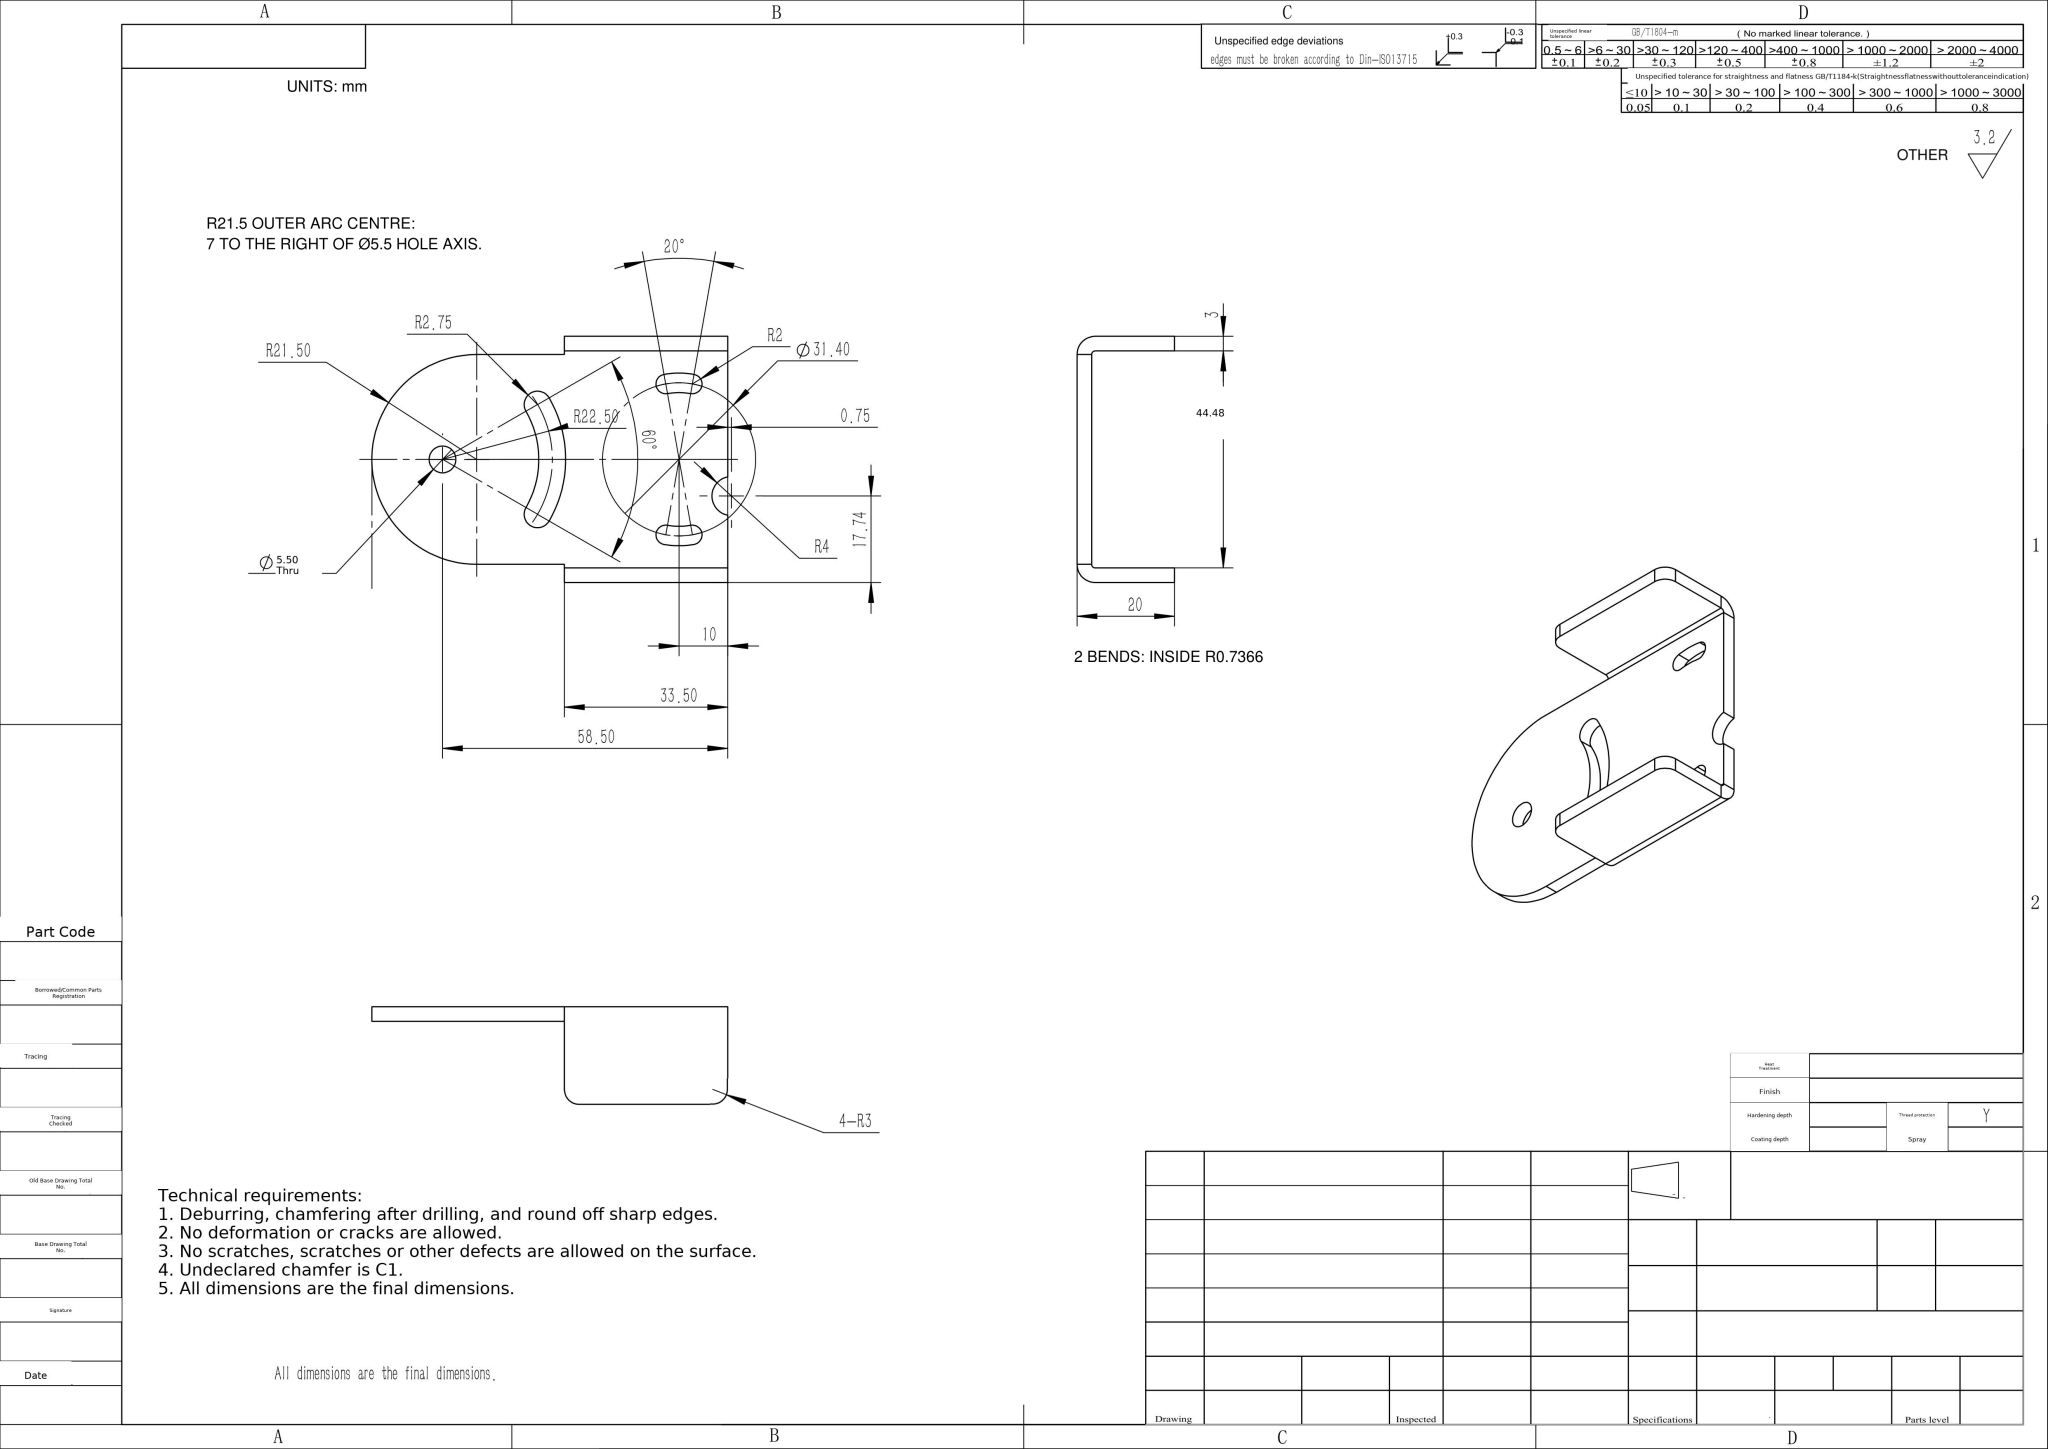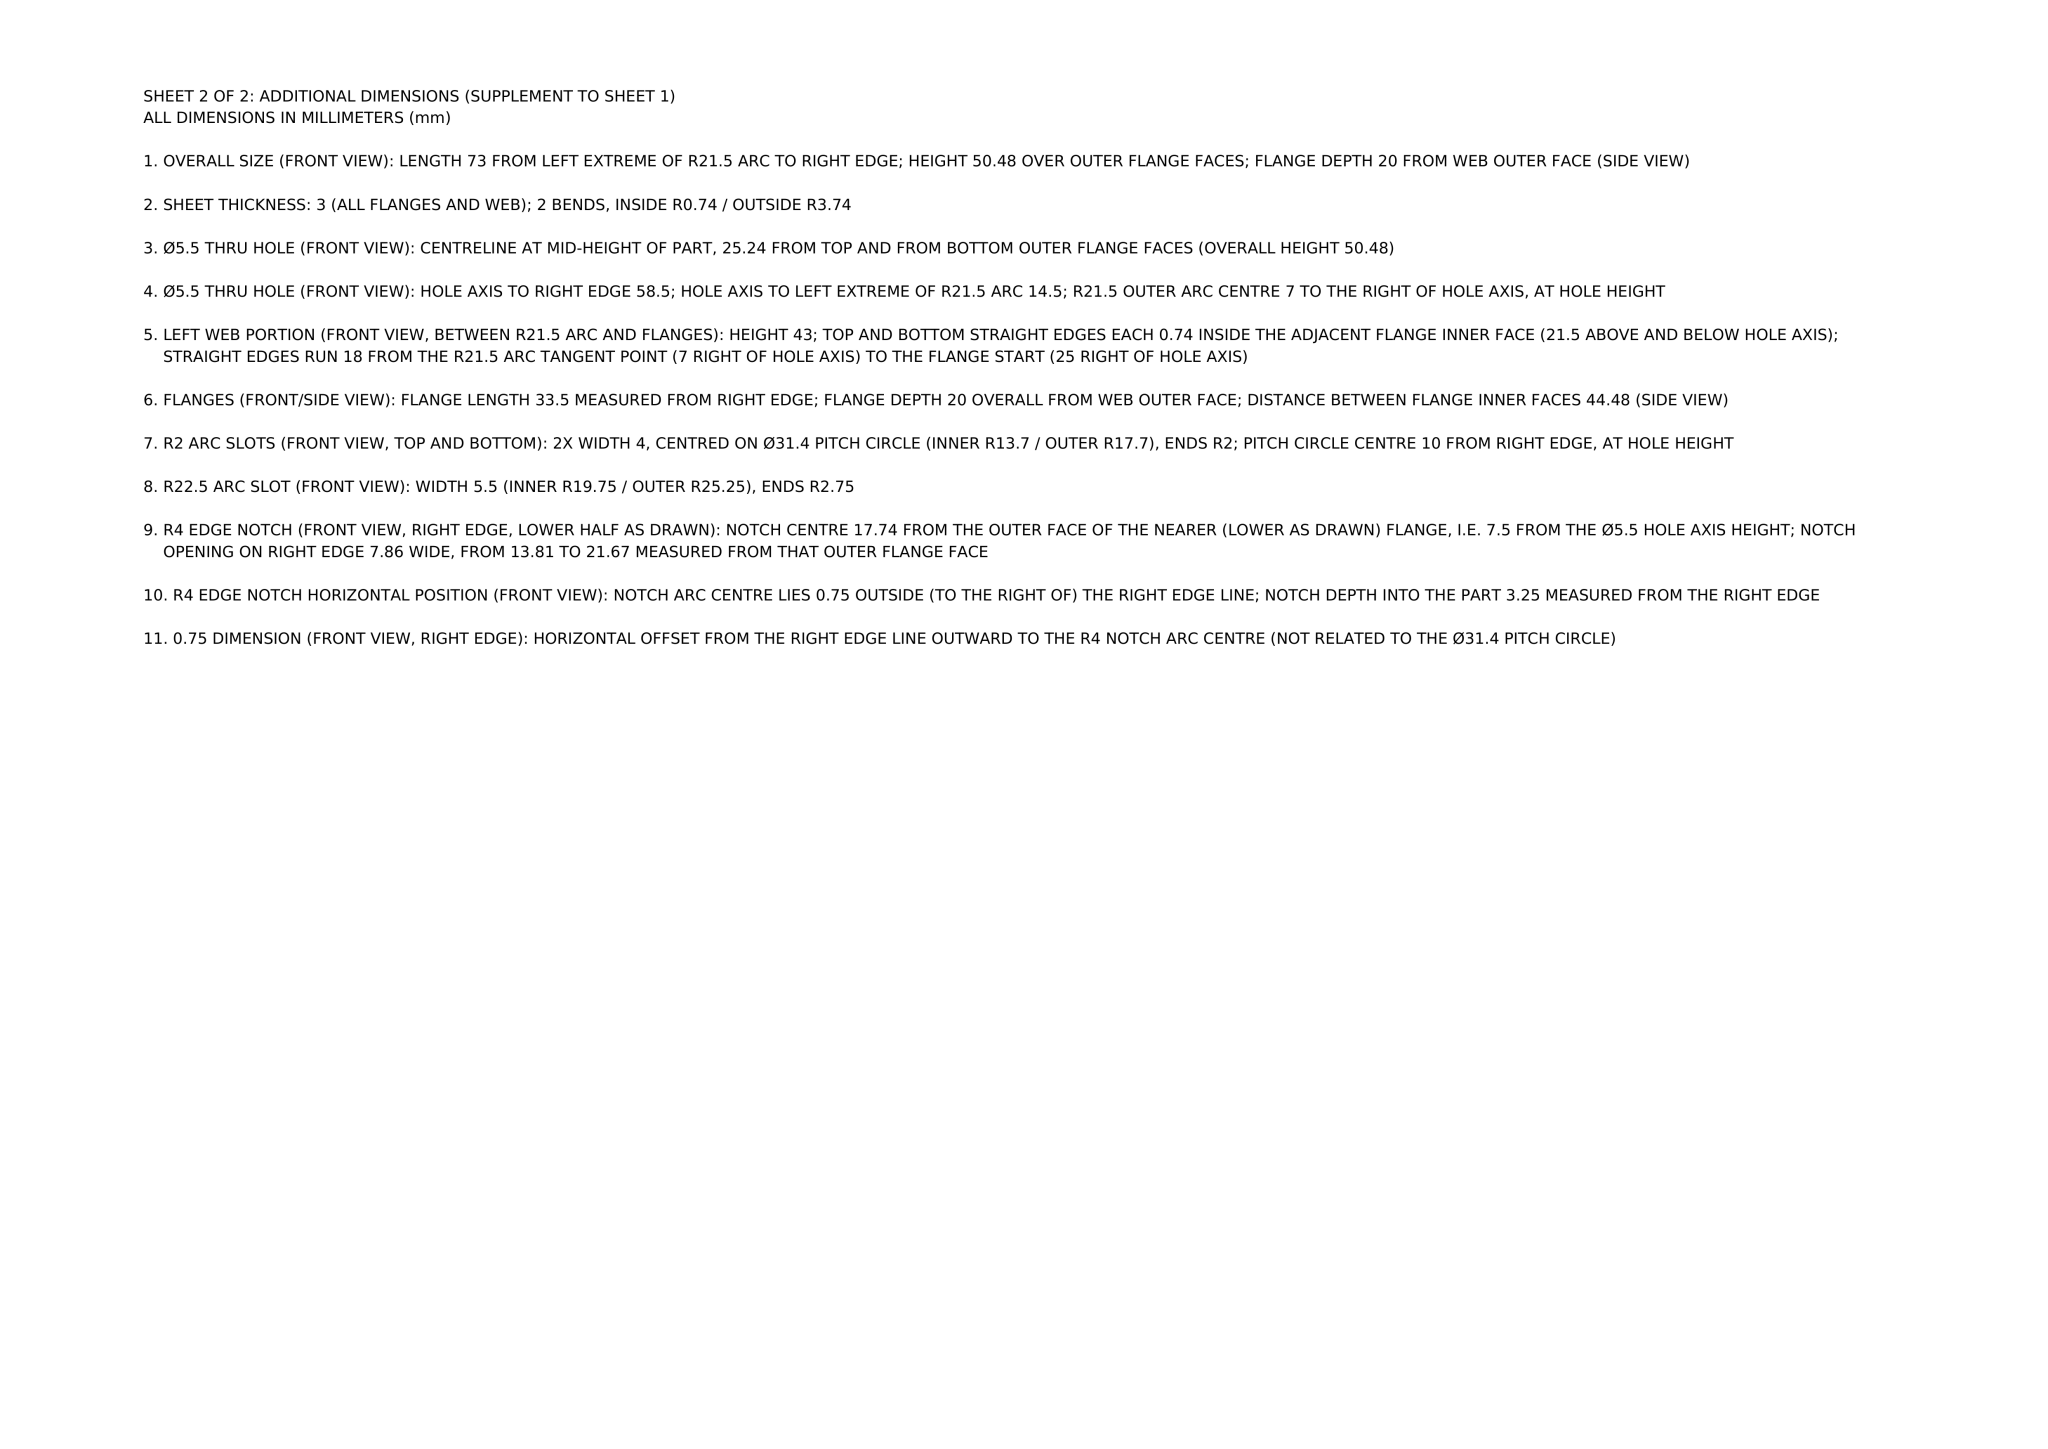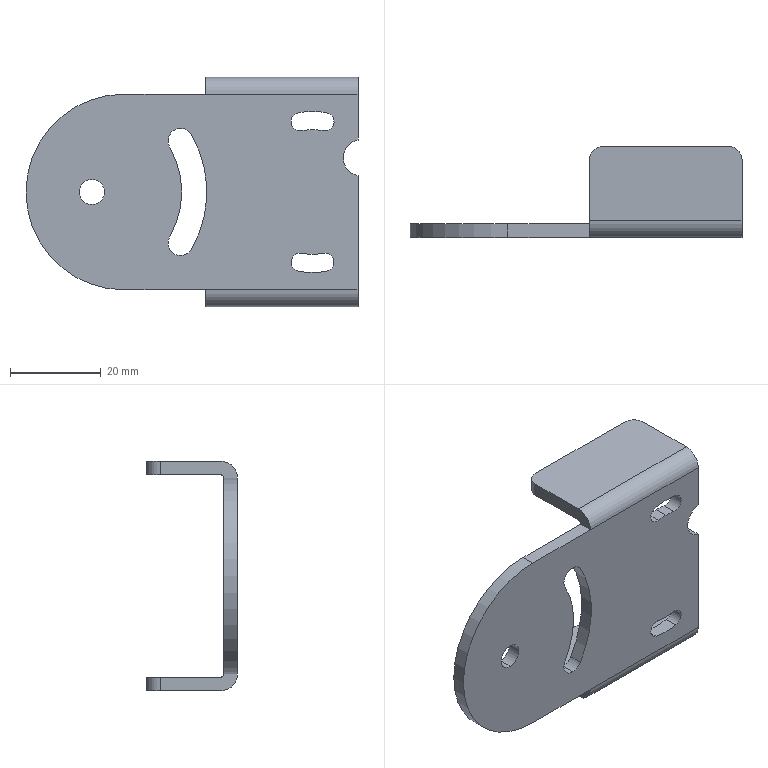Part | NX | mm | 1 solid | 47 faces | box 73 x 20 x 50.47 mm | volume 11978 mm3 | cylinder 29 | plane 18 | commonest cylinder face diameters 4 x6 5.5 x5 6 x4 27.4 x3 35.4 x3 7.473 x2 1.473 x2 43 x1